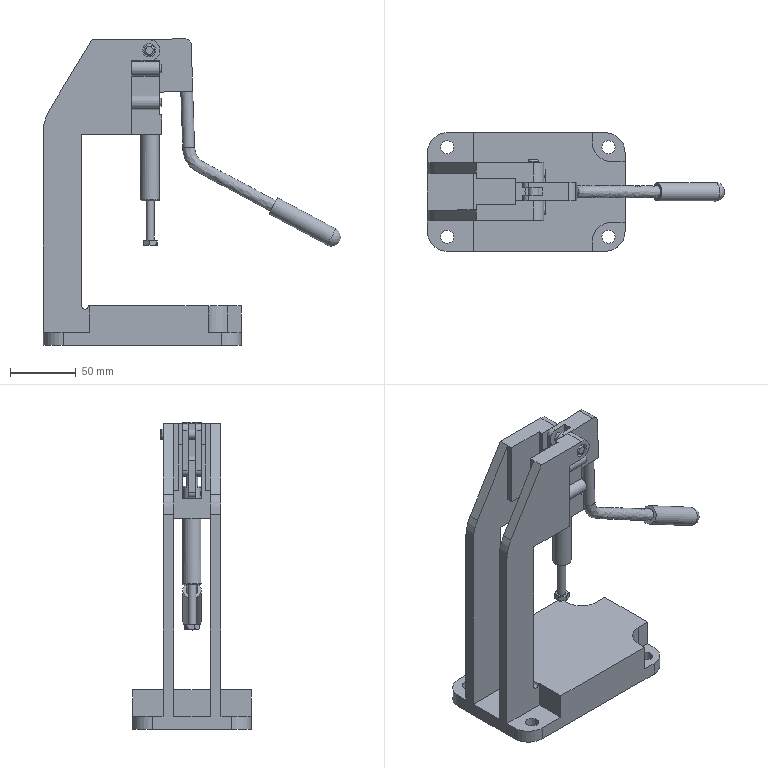Assembly | NX | mm | 8 component files | 9 solids | 167 faces | box 225.68 x 90 x 232.91 mm | volume 537446 mm3 | plane 103 | cylinder 50 | torus 10 | other 2 | spline 1 | sphere 1 | commonest cylinder face diameters 10 x11 5 x10 6 x6 30 x6 11 x4 8 x3 14 x3 7 x2
Bill of materials:
unnamed part 1 | 1 |  | Bent slender rod lever with a flat rectangular rounded-corner plate at one end and a larger-diameter cylindrical grip with rounded tip at the other end.
unnamed part 2 | 1 |  | Hex-head bolt-like part with a long, plain cylindrical shank and a chamfered/rounded end.
unnamed part 3 | 1 |  | Hollow cylindrical tube/pin with a slotted end forming two prongs, a cross hole through the prongs, and a slight step in outer diameter near the slotted end.
unnamed part 4 | 1 |  | Plain solid cylindrical pin/rod with small edge rounds or chamfers at both ends.
unnamed part 5 | 1 |  | Link plate/bar shaped like an obround (stadium) with a through hole at each rounded end.
unnamed part 6 | 2 |  | Short solid cylindrical pin with generously rounded edges at both ends.
unnamed part 7 | 1 |  | C-shaped bracket/stand: rectangular base plate with rounded corners and four corner holes, a vertical twin-wall column, and an upper overhanging arm ending in two parallel lugs with cross holes and short pin-like bosses.
Mates:
1. fix | machine_base 1 component
2. touch align | machine_base 1 face | handle 1 face
3. touch align | handle 1 face | link 1 face
4. touch align | handle 1 face | link 1 face
5. touch align | Centre_rod 1 face | machine_base 1 face
6. touch align | Centre_rod 1 face | link 1 face
7. touch align | bolt 1 face | Centre_rod 1 face
8. touch align | M8 1 face | machine_base 1 face
9. touch align | M8 1 face | machine_base 1 face
10. touch align | M5 2 face | handle 1 face
11. touch align | M5 2 face | handle 1 face
12. touch align | M5 1 face | Centre_rod 1 face
13. touch align | M5 1 face | Centre_rod 1 face
14. touch align | handle 1 face | machine_base 1 face